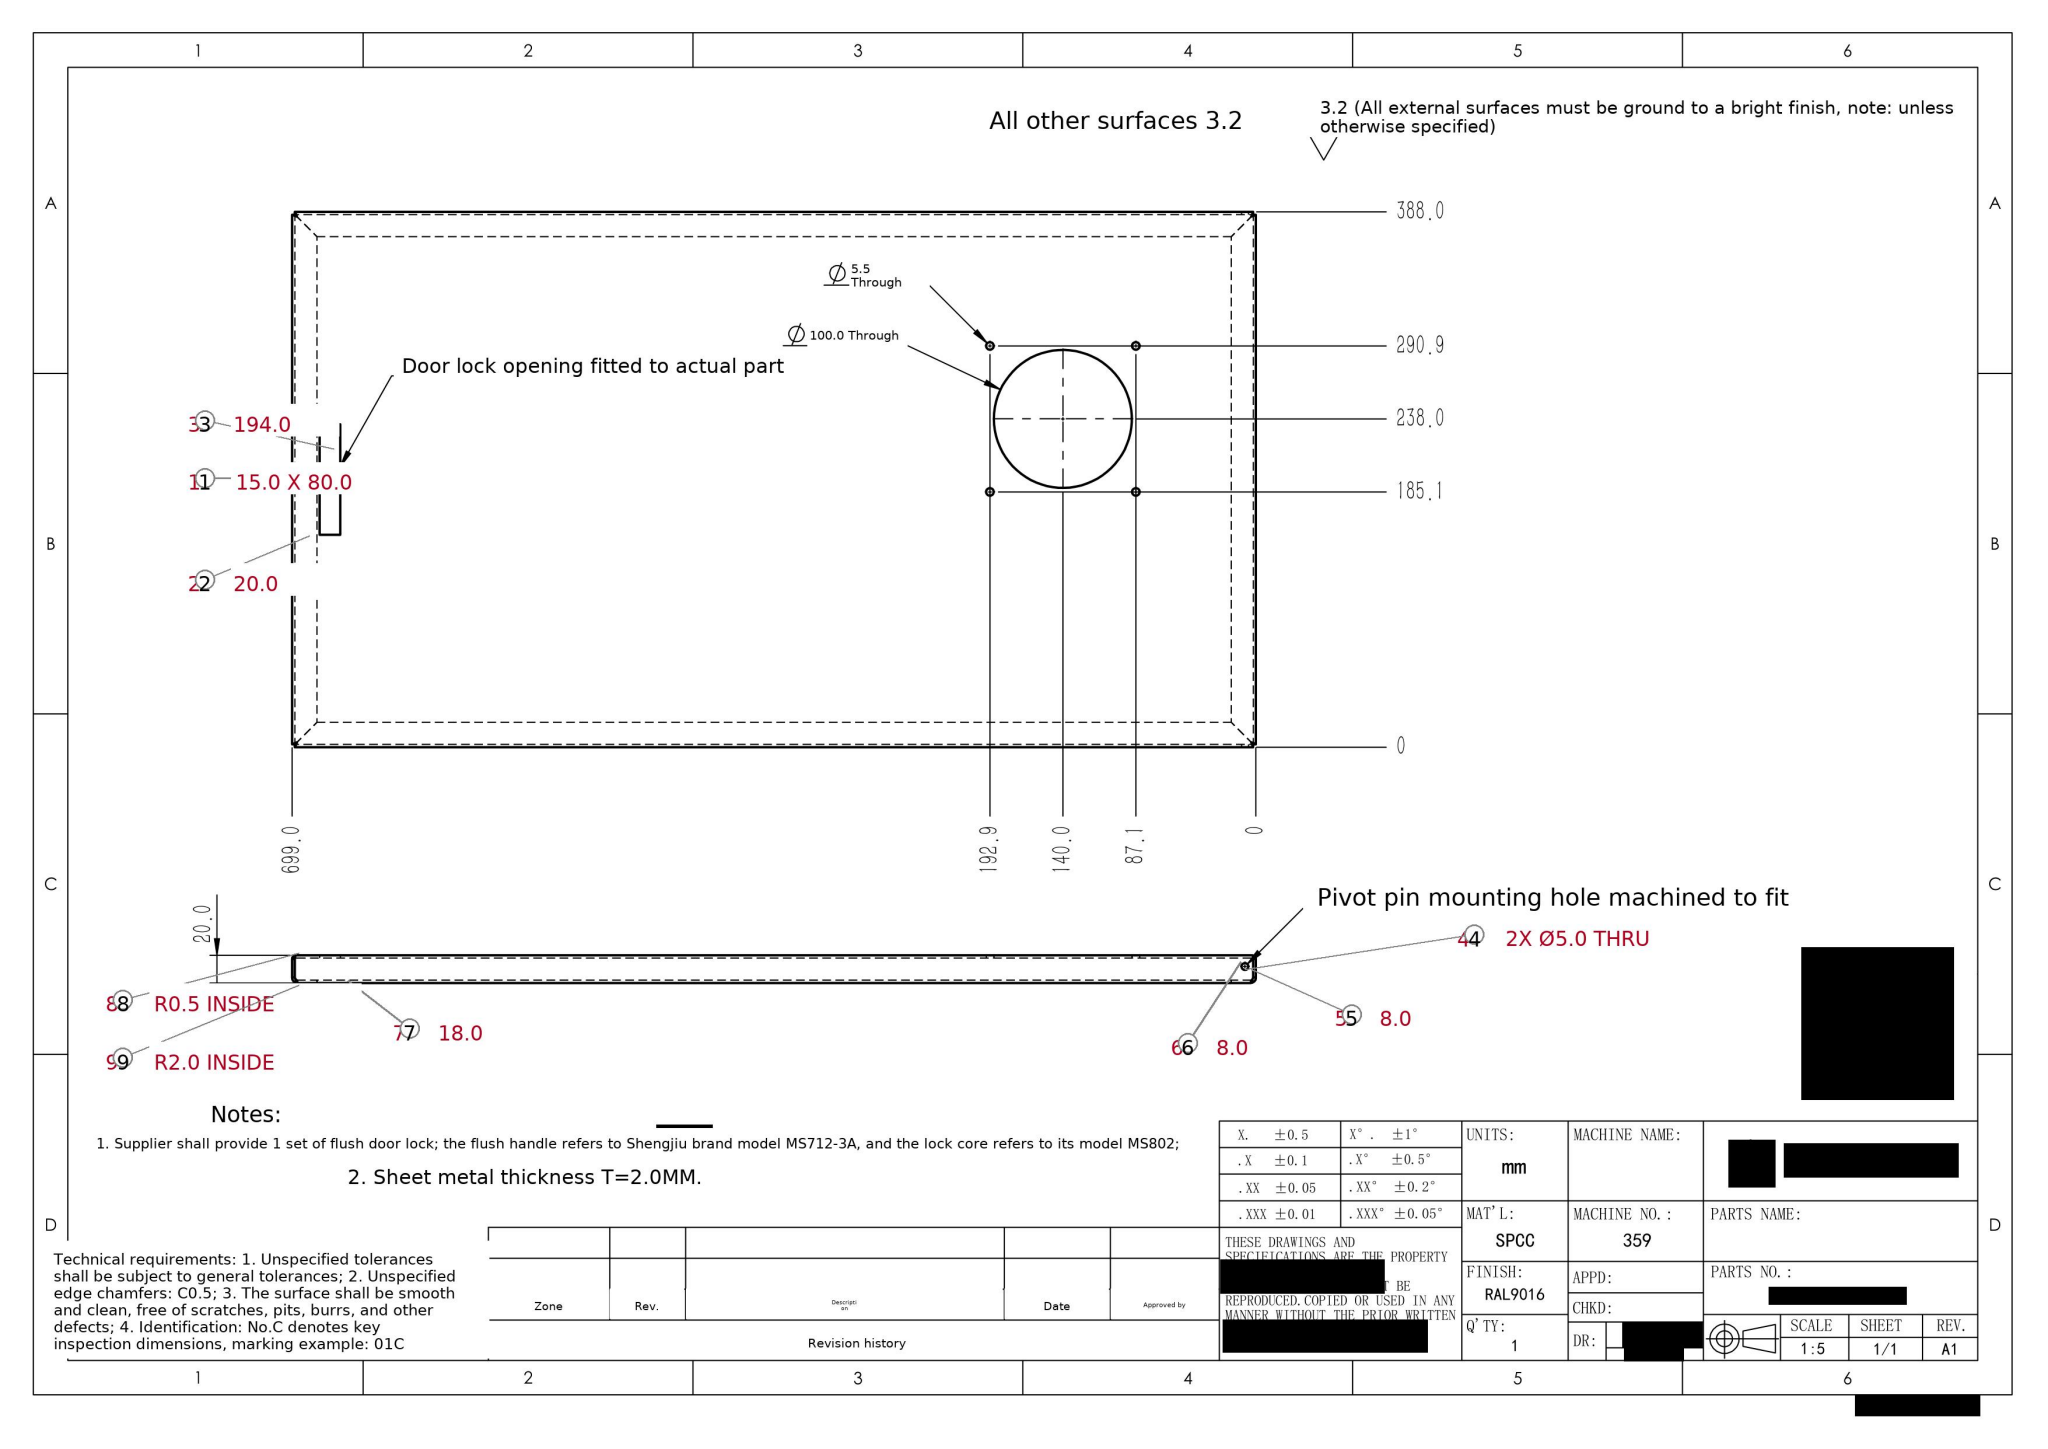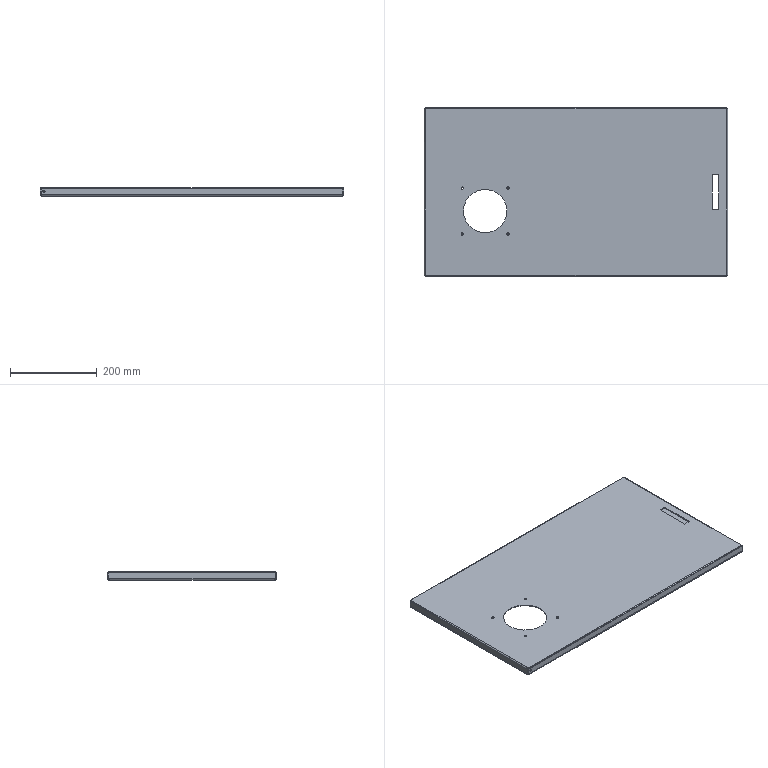Part | SolidWorks | mm | 1 solid | 88 faces | box 699 x 388 x 20 mm | volume 660287 mm3 | plane 42 | cylinder 30 | spline 16 | commonest cylinder face diameters 5.5 x8 5 x8 1 x4 8 x4 4 x4 100 x2